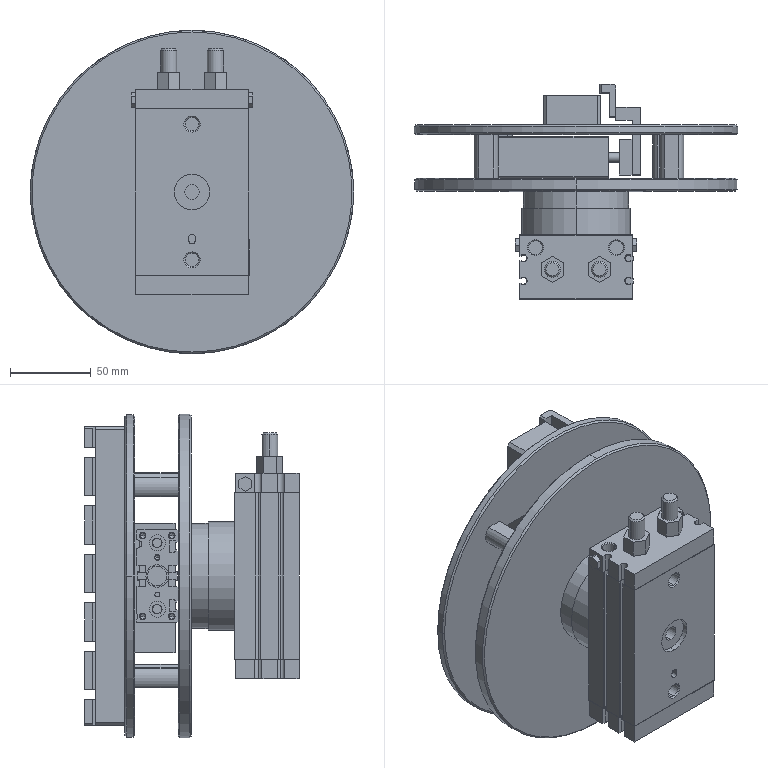Assembly | SolidWorks | mm | 13 component files | 13 solids | 839 faces | box 200 x 133 x 200 mm | volume 1043506 mm3 | plane 366 | cylinder 303 | cone 168 | spline 2 | commonest cylinder face diameters 4.917 x24 0.8 x20 28 x18 3 x18 6 x18 4 x17 4.6 x16 3.242 x16
Bill of materials:
Inline-H010-1 | 1 |  | Rectangular block body with two stepped cylindrical studs, each with a hexagonal collar, sticking out of one end face; grooves run along its length and it has through holes in the faces.
Inline-H010-2 | 1 |  | Short stepped cylindrical disc with a small central through bore.
Inline-H010-H01-001K | 1 |  | Thin flat circular disc with no holes.
Inline-H010-H01-002K | 1 |  | Narrow rectangular bar with a row of six equally spaced round through holes. One long edge has a series of small rectangular notches.
Inline-H010-H01160308-003K | 1 |  | Thin flat circular disc with two parallel rectangular through slots of slightly different sizes.
Inline-H010-H01160308-004K | 4 |  | Elongated cylindrical sleeve with a central through bore and two parallel flats machined along its length.
Inline-H010-H01160308-005K | 1 |  | Thin L-shaped (angle) plate with a short return flange along one edge.
Inline-H010-H01160308-006K | 1 |  | Long thin strip with an L-shaped end profile. One edge has a row of small, evenly spaced rectangular notches.
Inline-H010-TCL12x40SCylinder | 1 |  | Prismatic extruded profile with several longitudinal T-slot-like grooves on its sides. Its end face shows three axial bores, and a broad face has transverse through holes.
Inline-H010-TCL12x40SSteelBallGuide | 1 |  | Rectangular end plate holding two long parallel round rods and a shorter central rod, which ends in a larger cylindrical boss.
Mates:
1. coincident | Inline-H010-H01-001K-1 plane at (29.082, -10.032, 139.665) dir (1, 0, 0) | Inline-H010-H01-002K-1 plane at (29.082, 35.968, 139.665) dir (-1, 0, 0)
2. coincident | Inline-H010-H01-001K-1 plane at (29.082, -10.032, 139.665) dir (0, 0, -1) | Inline-H010-H01-002K-1 plane at (29.082, 35.968, 139.665) dir (0, 0, -1)
3. coincident | Inline-H010-A_EMSQA30A-A96(0)-1/Inline-H010-2-1 face at (29.082, -14.032, 139.665) dir (0, 1, 0) | Inline-H010-H01-001K-1 face at (29.082, -14.032, 139.665) dir (0, -1, 0)
4. concentric | Inline-H010-A_EMSQA30A-A96(0)-1/Inline-H010-2-1 face at (29.082, -24.532, 139.665) dir (0, -1, 0) r 32.5 | Inline-H010-H01-001K-1 face at (29.082, -14.032, 139.665) dir (0, 1, 0) r 100
5. coincident | Inline-H010-H01-002K-1 face at (29.082, 26.968, 139.665) dir (0, -1, 0) | Inline-H010-H01160308-003K-1 face at (29.082, 26.968, 139.665) dir (0, 1, 0)
6. concentric | Inline-H010-H01-001K-1 face at (29.082, -14.032, 139.665) dir (0, 1, 0) r 100 | Inline-H010-H01160308-003K-1 face at (29.082, 20.968, 139.665) dir (0, 1, 0) r 100
7. coincident | Inline-H010-H01-001K-1 face at (29.082, -6.032, 139.665) dir (0, 1, 0) | Inline-H010-TCL12x40S_0_+_CS1-G-1-3/Inline-H010-TCL12x40SCylinder-1 face at (48.982, -6.032, 132.665) dir (0, -1, 0)
8. parallel | Inline-H010-H01-002K-1 face at (44.082, 44.968, 47.165) dir (1, 0, 0) | Inline-H010-H01160308-003K-1 face at (44.11, 16.968, 80.091) dir (1, 0, 0)
9. coincident | Inline-H010-H01160308-003K-1 plane at (29.082, 23.968, 139.665) dir (0, 0, 1) | Inline-H010-TCL12x40S_0_+_CS1-G-1-3/Inline-H010-TCL12x40SCylinder-1 plane at (48.982, 6.968, 139.665) dir (0, 0, 1)
10. coincident | Inline-H010-H01-001K-1 face at (29.082, -6.032, 139.665) dir (0, 1, 0) | Inline-H010-H01160308-004K-1 face at (-19.023, -6.032, 194.941) dir (0, -1, 0)
11. coincident | Inline-H010-H01-001K-1 face at (29.082, -6.032, 139.665) dir (0, 1, 0) | Inline-H010-H01160308-004K-2 face at (95.77, -6.032, 197.578) dir (0, -1, 0)
12. coincident | Inline-H010-H01160308-004K-1 face at (-41.654, 8.804, 200.423) dir (-0.02297, 0, 0.9997) | Inline-H010-H01160308-004K-2 face at (73.138, 8.804, 203.06) dir (-0.02297, 0, 0.9997)
13. coincident | Inline-H010-H01-001K-1 face at (29.082, -6.032, 139.665) dir (0, 1, 0) | Inline-H010-H01160308-004K-3 face at (-10.414, -6.032, 76.826) dir (0, -1, 0)
14. coincident | Inline-H010-H01-001K-1 face at (29.082, -6.032, 139.665) dir (0, 1, 0) | Inline-H010-H01160308-004K-4 face at (91.486, -6.032, 79.167) dir (0, -1, 0)
15. parallel | Inline-H010-H01160308-004K-1 face at (-41.654, 8.804, 200.423) dir (-0.02297, 0, 0.9997) | Inline-H010-H01160308-004K-3 face at (-33.046, 8.804, 82.308) dir (-0.02297, 0, 0.9997)
16. coincident | Inline-H010-H01160308-004K-3 face at (-33.046, 8.804, 82.308) dir (-0.02297, 0, 0.9997) | Inline-H010-H01160308-004K-4 face at (68.854, 8.804, 84.649) dir (-0.02297, 0, 0.9997)
17. coincident | Inline-H010-H01160308-003K-1 face at (29.082, 20.968, 139.665) dir (0, -1, 0) | Inline-H010-H01160308-004K-2 face at (88.272, 20.968, 197.406) dir (0, 1, 0)
18. coincident | Inline-H010-TCL12x40S_0_+_CS1-G-1-3/Inline-H010-TCL12x40SSteelBallGuide-1 face at (63.768, 6.968, 139.665) dir (1, 0, 0) | Inline-H010-H01160308-005K-1 face at (63.768, 29.968, 92.262) dir (-1, 0, 0)
19. coincident | Inline-H010-TCL12x40S_0_+_CS1-G-1-3/Inline-H010-TCL12x40SSteelBallGuide-1 face at (63.768, -4.032, 167.665) dir (0, -1, 0) | Inline-H010-H01160308-005K-1 face at (63.768, -4.032, 92.262) dir (0, -1, 0)
20. coincident | Inline-H010-H01160308-005K-1 face at (53.768, 37.968, 92.262) dir (-1, 0, 0) | Inline-H010-H01160308-006K-1 face at (53.768, 51.968, 232.165) dir (1, 0, 0)
21. coincident | Inline-H010-H01-002K-1 face at (44.082, 44.968, 232.165) dir (0, 0, 1) | Inline-H010-H01160308-006K-1 face at (-6.88, 51.968, 232.165) dir (0, 0, 1)
22. distance | Inline-H010-H01160308-005K-1 face at (53.768, 29.968, 92.262) dir (0, -1, 0) | Inline-H010-H01160308-006K-1 face at (53.768, 31.968, 232.165) dir (0, -1, 0)
23. concentric | Inline-H010-TCL12x40SCylinder-1 face at (50.279, -32.029, -8.689) dir (1, 0, 0) r 5 | Inline-H010-TCL12x40SSteelBallGuide-1 face at (27.869, -32.029, -8.689) dir (1, 0, 0) r 3